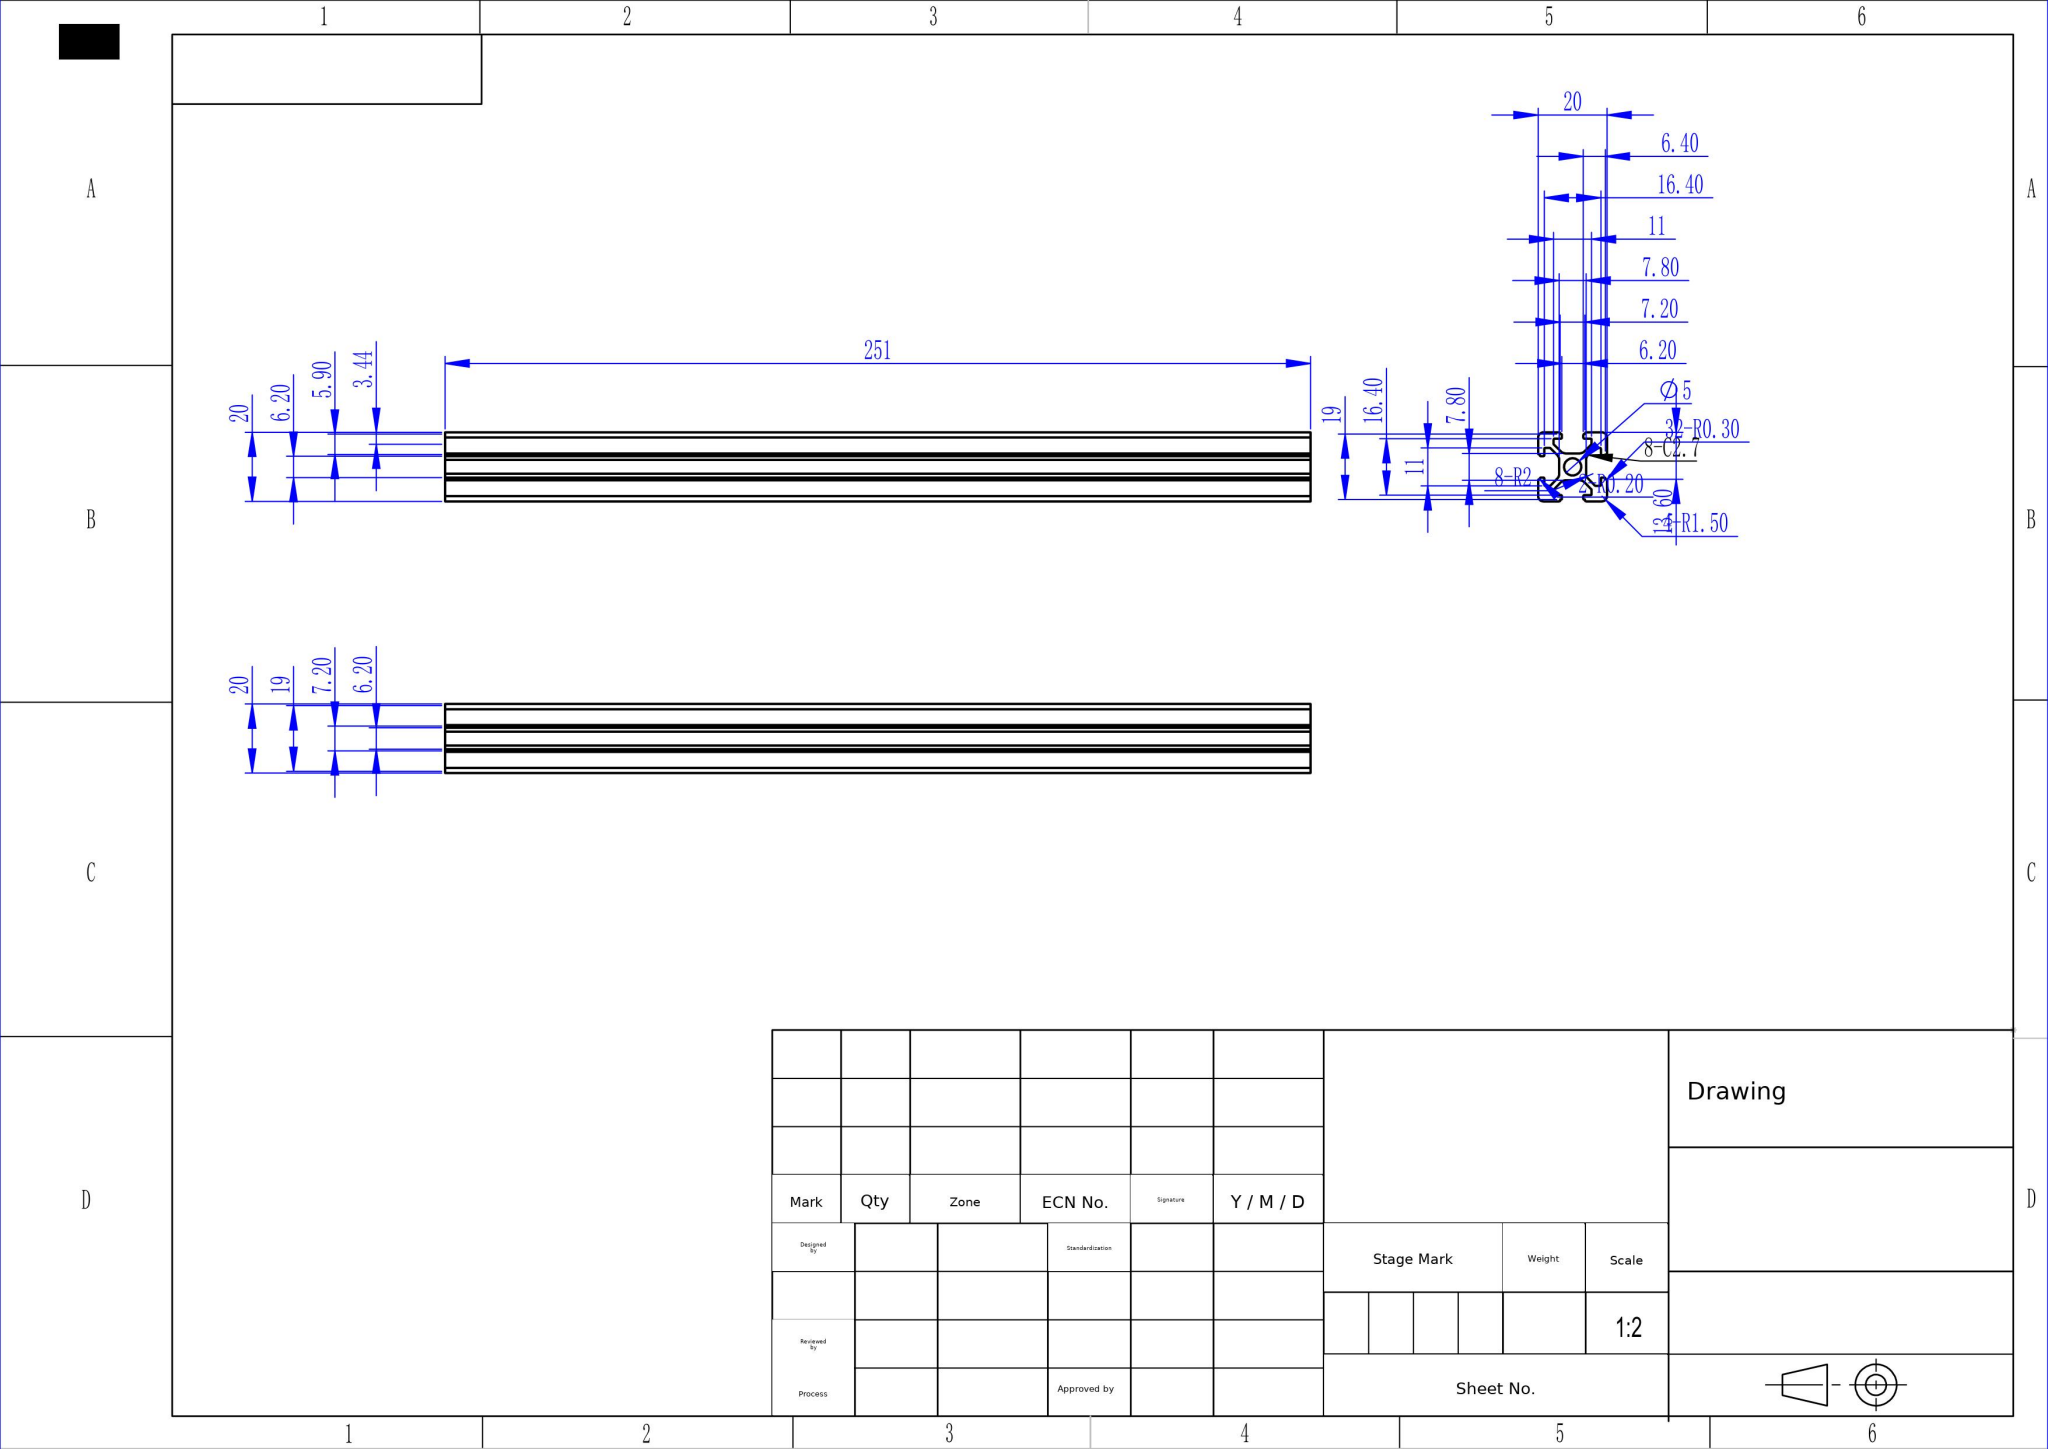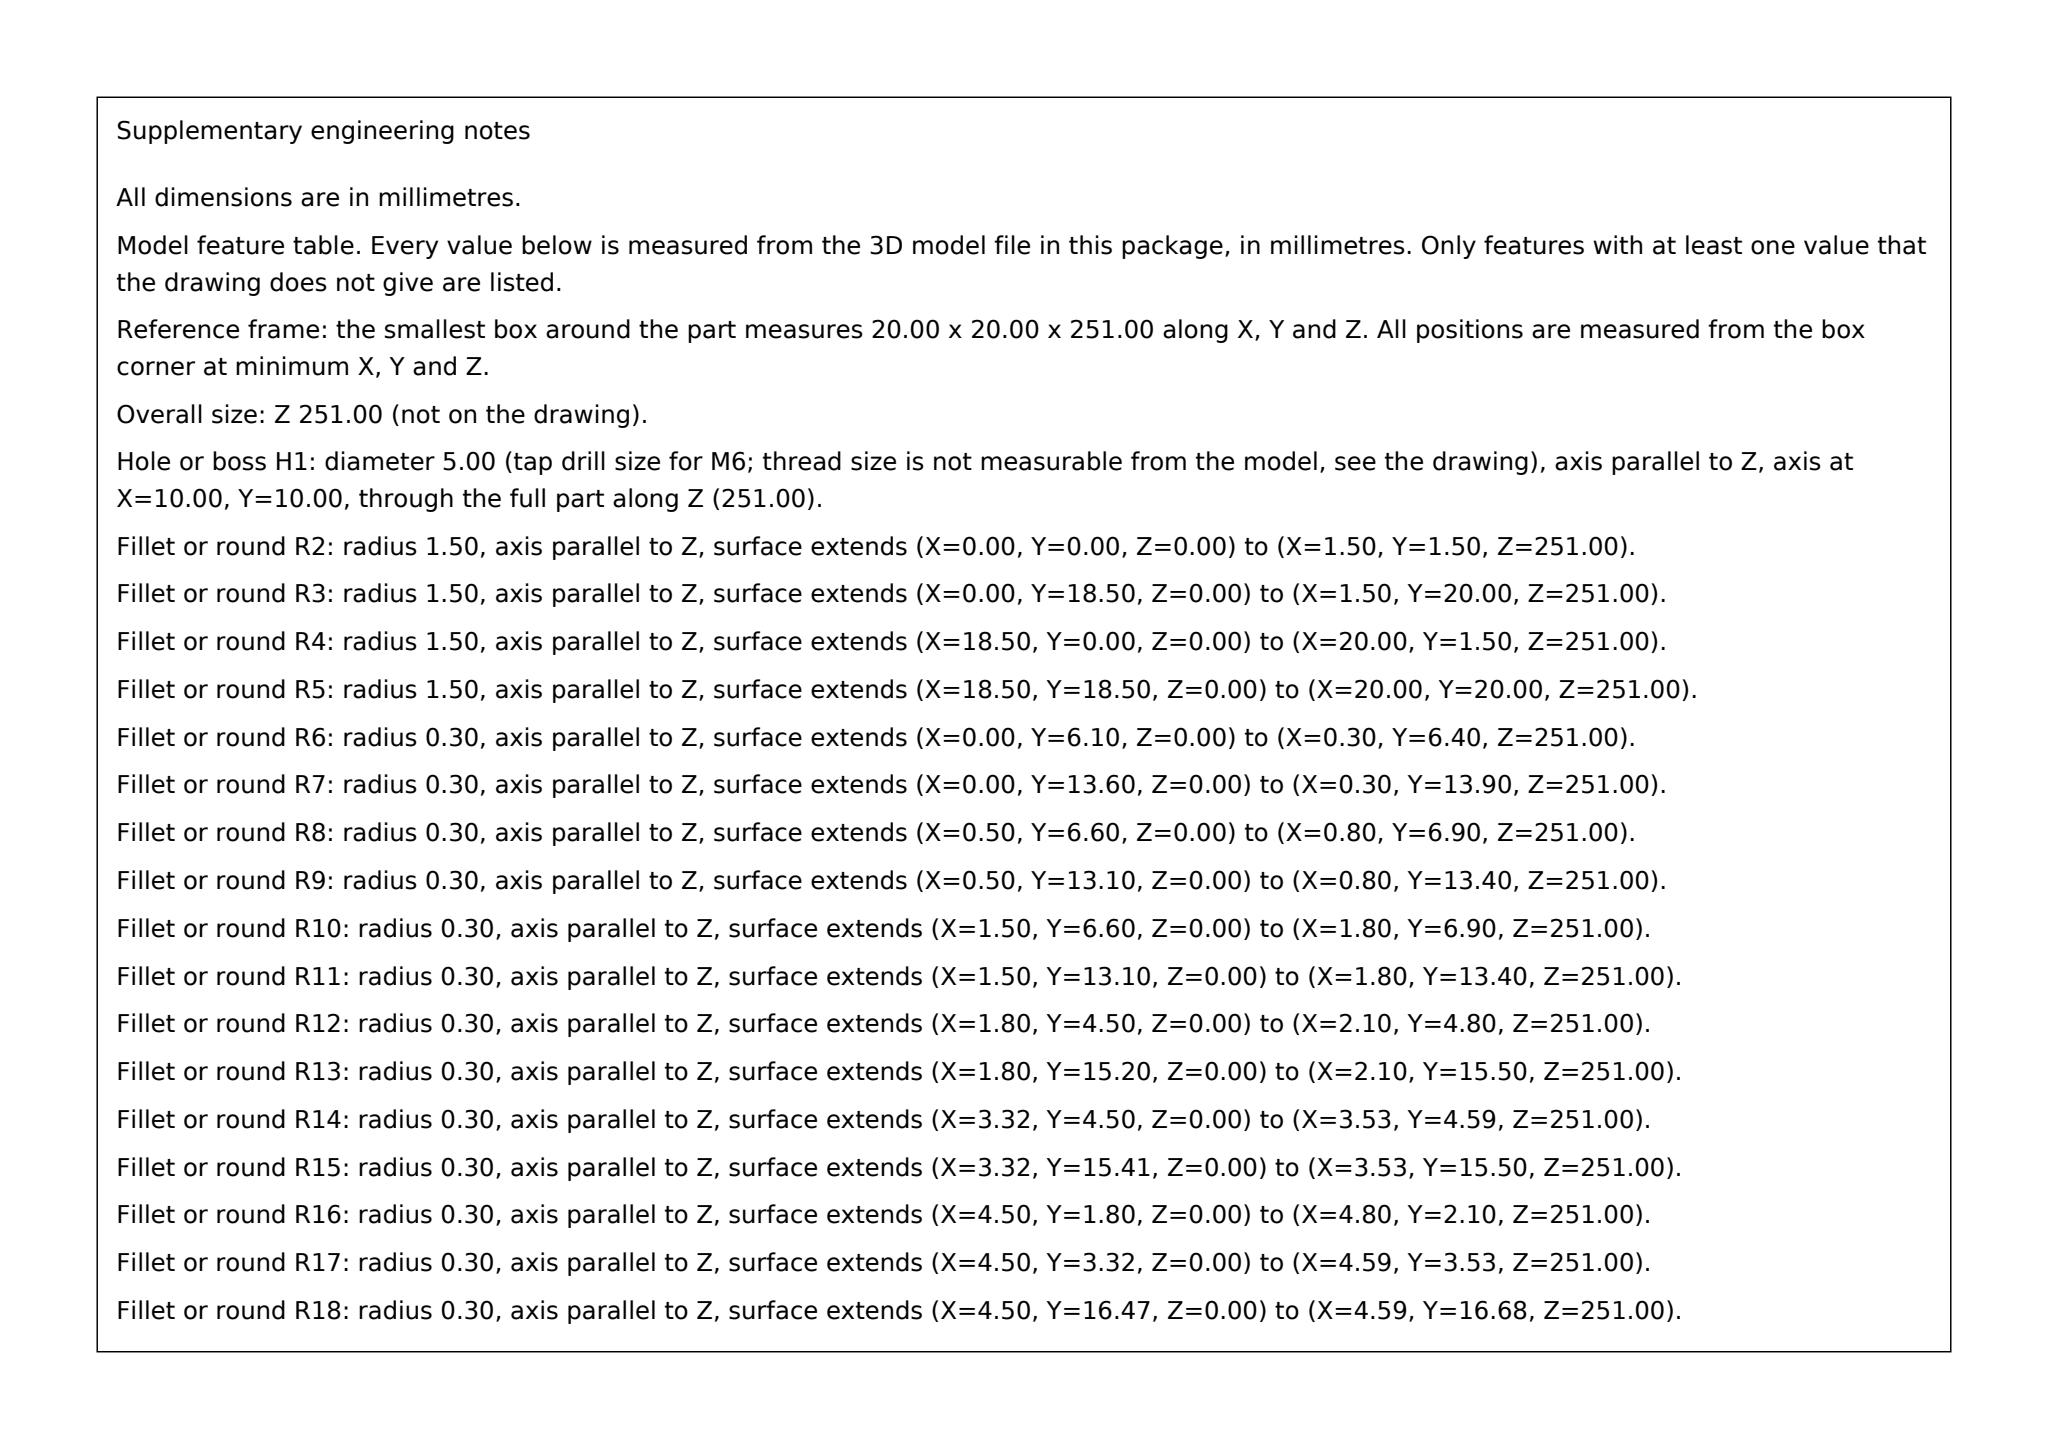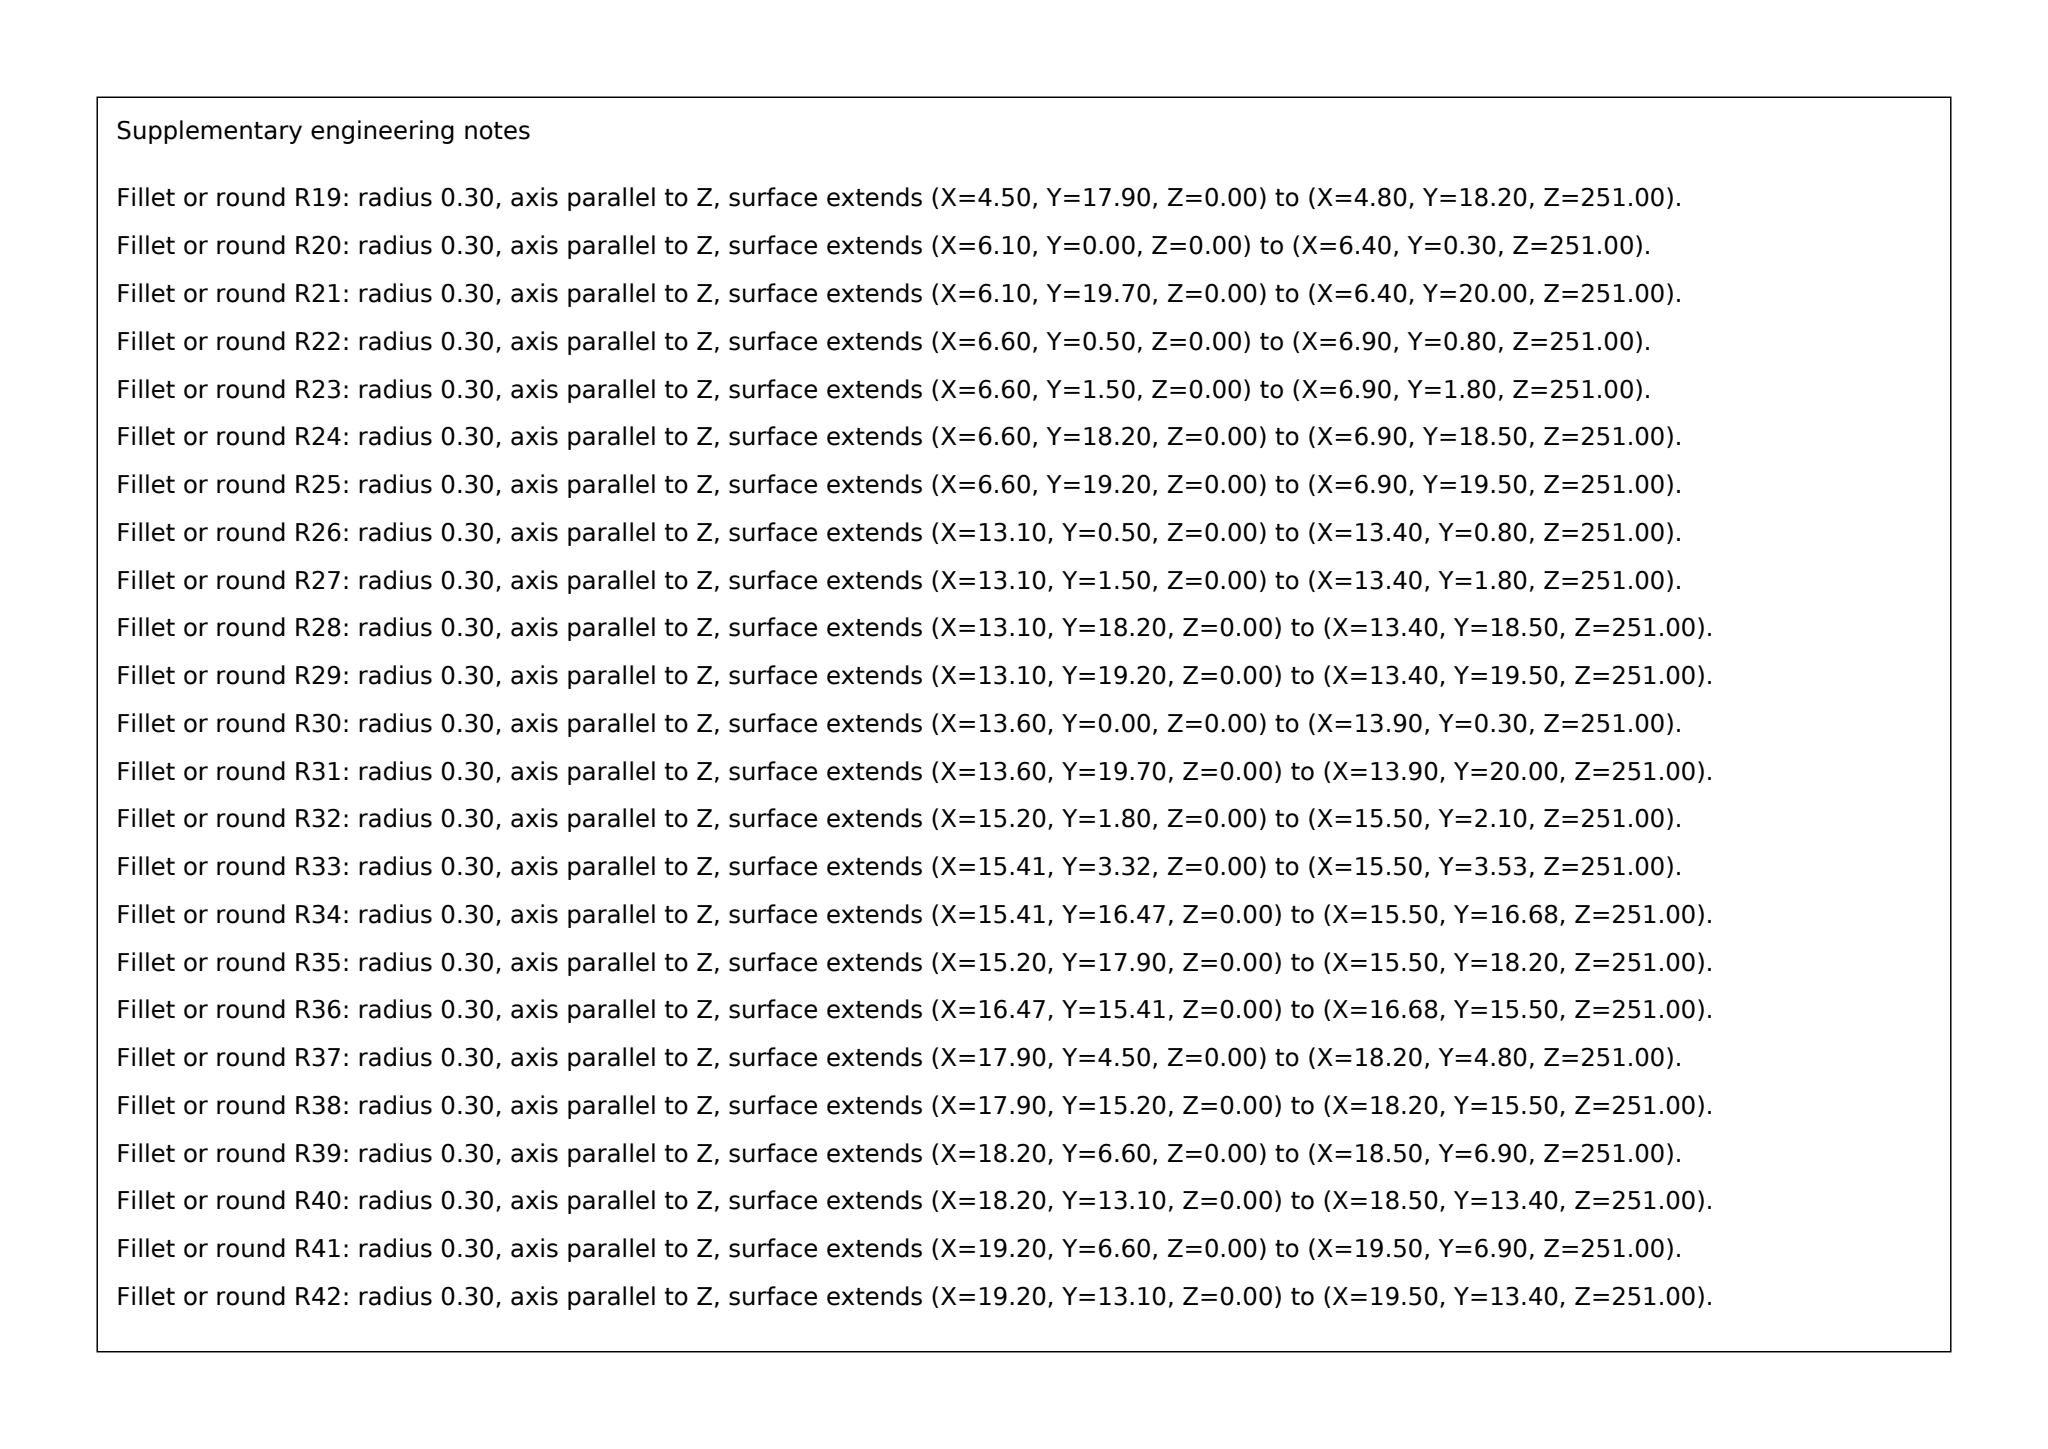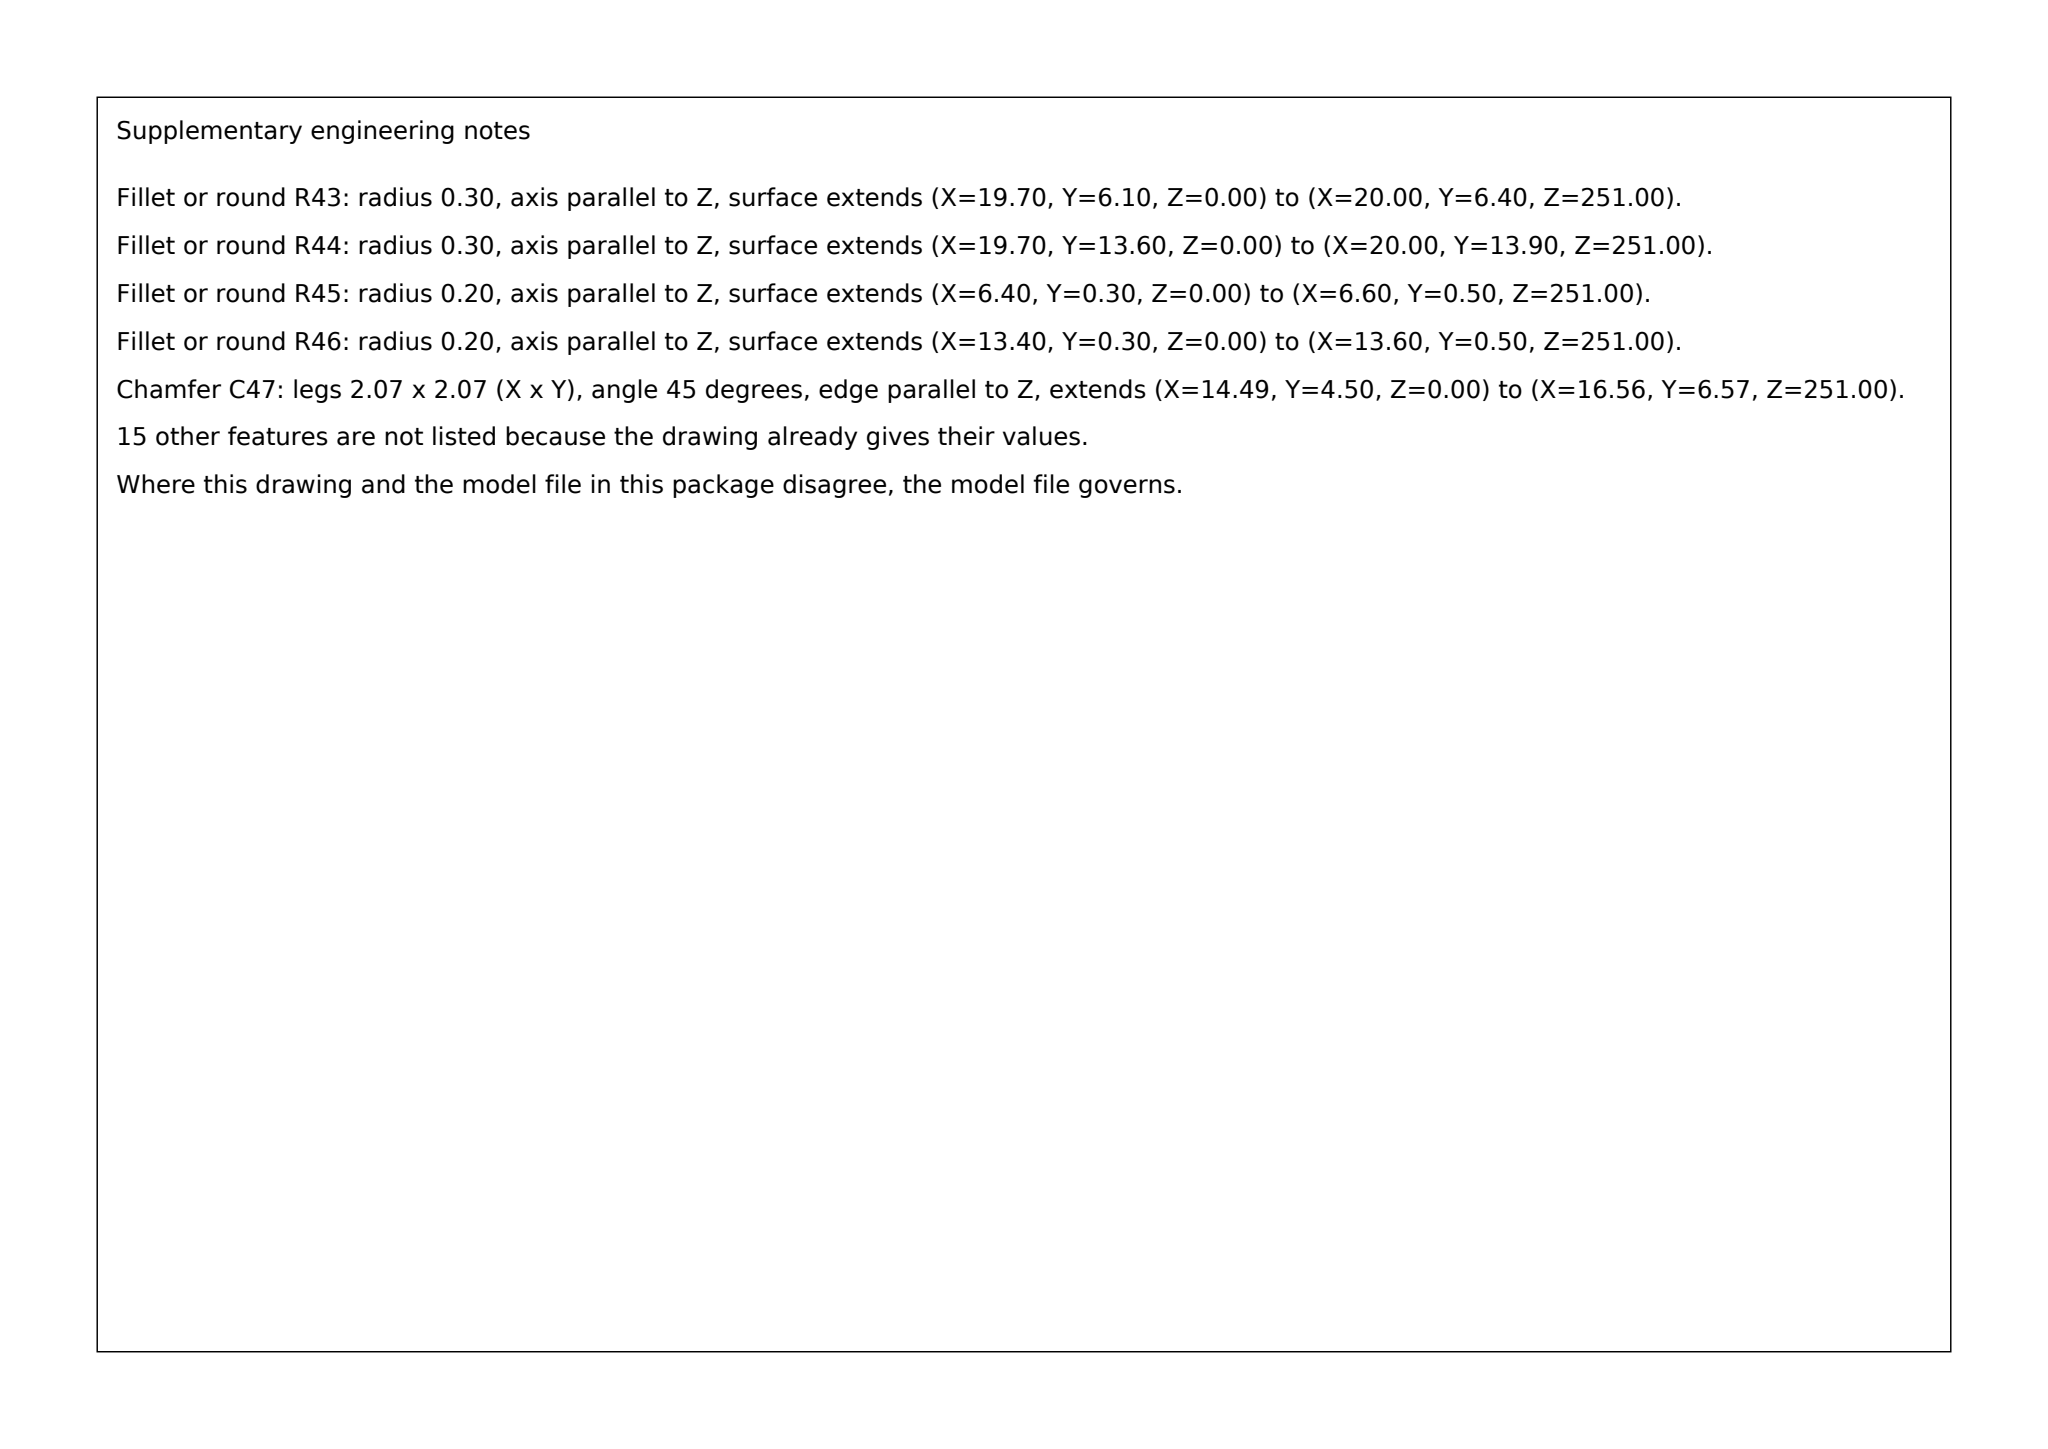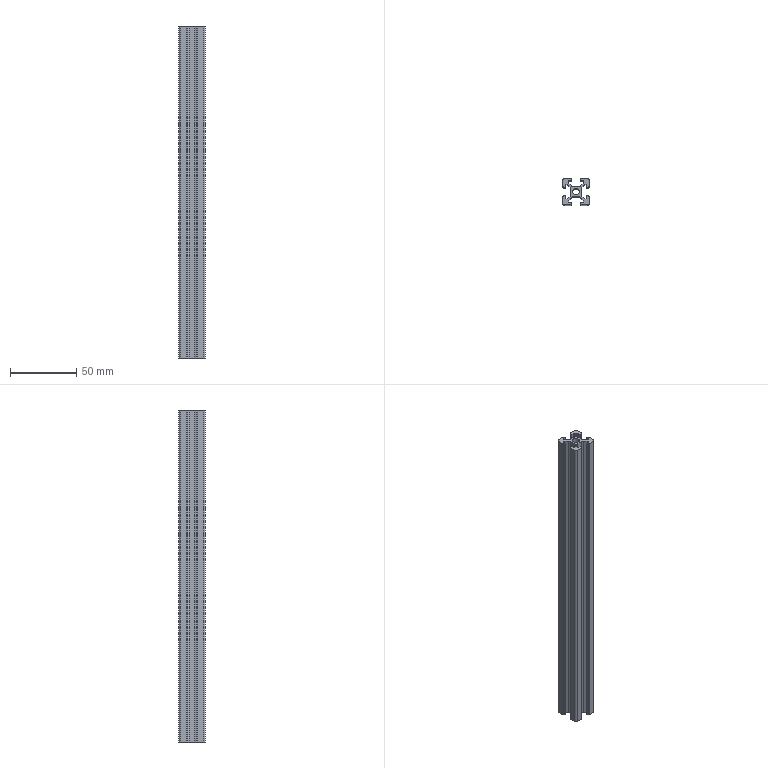Part | SolidWorks | mm | 1 solid | 113 faces | box 20 x 20 x 251 mm | volume 43001 mm3 | plane 58 | cylinder 55 | commonest cylinder face diameters 0.6 x39 4 x8 3 x4 5 x2 0.4 x2
build123d program:
from build123d import *

# Parameters (mm, degrees)
SKETCH1_R           = 2.5
BOSS_EXTRUDE1_DEPTH = 251


with BuildPart() as part:
    # Sketch1 → Boss-Extrude1 (new body)
    with BuildSketch(Plane(origin=(0, 0, 0), x_dir=(-1, 0, 0), z_dir=(0, 0, -1))):
        with BuildLine():
            Line((-5845.236, 2818.35), (-5845.236, 2820.15))
            ThreePointArc((-5845.236, 2820.15), (-5845.323, 2820.362), (-5845.536, 2820.45))
            Line((-5845.536, 2820.45), (-5846.236, 2820.45))
            ThreePointArc((-5846.236, 2820.45), (-5846.448, 2820.362), (-5846.536, 2820.15))
            Line((-5846.536, 2820.15), (-5846.536, 2819.95))
            Line((-5846.536, 2819.95), (-5846.736, 2819.95))
            ThreePointArc((-5846.736, 2819.95), (-5846.948, 2819.862), (-5847.036, 2819.65))
            Line((-5847.036, 2819.65), (-5847.036, 2815.05))
            ThreePointArc((-5847.036, 2815.05), (-5846.596, 2813.989), (-5845.536, 2813.55))
            Line((-5845.536, 2813.55), (-5840.936, 2813.55))
            ThreePointArc((-5840.936, 2813.55), (-5840.723, 2813.638), (-5840.636, 2813.85))
            ThreePointArc((-5840.636, 2813.85), (-5840.577, 2813.991), (-5840.436, 2814.05))
            ThreePointArc((-5840.436, 2814.05), (-5840.223, 2814.138), (-5840.136, 2814.35))
            Line((-5840.136, 2814.35), (-5840.136, 2815.05))
            ThreePointArc((-5840.136, 2815.05), (-5840.223, 2815.262), (-5840.436, 2815.35))
            Line((-5840.436, 2815.35), (-5842.236, 2815.35))
            ThreePointArc((-5842.236, 2815.35), (-5842.448, 2815.438), (-5842.536, 2815.65))
            Line((-5842.536, 2815.65), (-5842.536, 2816.865))
            ThreePointArc((-5842.536, 2816.865), (-5842.513, 2816.98), (-5842.448, 2817.077))
            Line((-5842.448, 2817.077), (-5840.461, 2819.064))
            ThreePointArc((-5840.461, 2819.064), (-5839.812, 2819.498), (-5839.046, 2819.65))
            Line((-5839.046, 2819.65), (-5835.025, 2819.65))
            ThreePointArc((-5835.025, 2819.65), (-5834.259, 2819.498), (-5833.61, 2819.064))
            Line((-5833.61, 2819.064), (-5831.623, 2817.077))
            ThreePointArc((-5831.623, 2817.077), (-5831.558, 2816.98), (-5831.536, 2816.865))
            Line((-5831.536, 2816.865), (-5831.536, 2815.65))
            ThreePointArc((-5831.536, 2815.65), (-5831.623, 2815.438), (-5831.836, 2815.35))
            Line((-5831.836, 2815.35), (-5833.636, 2815.35))
            ThreePointArc((-5833.636, 2815.35), (-5833.848, 2815.262), (-5833.936, 2815.05))
            Line((-5833.936, 2815.05), (-5833.936, 2814.35))
            ThreePointArc((-5833.936, 2814.35), (-5833.848, 2814.138), (-5833.636, 2814.05))
            ThreePointArc((-5833.636, 2814.05), (-5833.494, 2813.991), (-5833.436, 2813.85))
            ThreePointArc((-5833.436, 2813.85), (-5833.348, 2813.638), (-5833.136, 2813.55))
            Line((-5833.136, 2813.55), (-5828.536, 2813.55))
            ThreePointArc((-5828.536, 2813.55), (-5827.475, 2813.989), (-5827.036, 2815.05))
            Line((-5827.036, 2815.05), (-5827.036, 2819.65))
            ThreePointArc((-5827.036, 2819.65), (-5827.123, 2819.862), (-5827.336, 2819.95))
            Line((-5827.336, 2819.95), (-5827.536, 2819.95))
            Line((-5827.536, 2819.95), (-5827.536, 2820.15))
            ThreePointArc((-5827.536, 2820.15), (-5827.623, 2820.362), (-5827.836, 2820.45))
            Line((-5827.836, 2820.45), (-5828.536, 2820.45))
            ThreePointArc((-5828.536, 2820.45), (-5828.748, 2820.362), (-5828.836, 2820.15))
            Line((-5828.836, 2820.15), (-5828.836, 2818.35))
            ThreePointArc((-5828.836, 2818.35), (-5828.923, 2818.138), (-5829.136, 2818.05))
            Line((-5829.136, 2818.05), (-5830.351, 2818.05))
            ThreePointArc((-5830.351, 2818.05), (-5830.465, 2818.073), (-5830.563, 2818.138))
            Line((-5830.563, 2818.138), (-5832.55, 2820.125))
            ThreePointArc((-5832.55, 2820.125), (-5832.983, 2820.774), (-5833.136, 2821.539))
            Line((-5833.136, 2821.539), (-5833.136, 2825.561))
            ThreePointArc((-5833.136, 2825.561), (-5832.983, 2826.326), (-5832.55, 2826.975))
            Line((-5832.55, 2826.975), (-5830.563, 2828.962))
            ThreePointArc((-5830.563, 2828.962), (-5830.465, 2829.027), (-5830.351, 2829.05))
            Line((-5830.351, 2829.05), (-5829.136, 2829.05))
            ThreePointArc((-5829.136, 2829.05), (-5828.923, 2828.962), (-5828.836, 2828.75))
            Line((-5828.836, 2828.75), (-5828.836, 2826.95))
            ThreePointArc((-5828.836, 2826.95), (-5828.748, 2826.738), (-5828.536, 2826.65))
            Line((-5828.536, 2826.65), (-5827.836, 2826.65))
            ThreePointArc((-5827.836, 2826.65), (-5827.623, 2826.738), (-5827.536, 2826.95))
            Line((-5827.536, 2826.95), (-5827.536, 2827.15))
            Line((-5827.536, 2827.15), (-5827.336, 2827.15))
            ThreePointArc((-5827.336, 2827.15), (-5827.123, 2827.238), (-5827.036, 2827.45))
            Line((-5827.036, 2827.45), (-5827.036, 2832.05))
            ThreePointArc((-5827.036, 2832.05), (-5827.475, 2833.11), (-5828.536, 2833.55))
            Line((-5828.536, 2833.55), (-5833.136, 2833.55))
            ThreePointArc((-5833.136, 2833.55), (-5833.348, 2833.462), (-5833.436, 2833.25))
            Line((-5833.436, 2833.25), (-5833.436, 2833.05))
            Line((-5833.436, 2833.05), (-5833.636, 2833.05))
            ThreePointArc((-5833.636, 2833.05), (-5833.848, 2832.962), (-5833.936, 2832.75))
            Line((-5833.936, 2832.75), (-5833.936, 2832.05))
            ThreePointArc((-5833.936, 2832.05), (-5833.848, 2831.838), (-5833.636, 2831.75))
            Line((-5833.636, 2831.75), (-5831.836, 2831.75))
            ThreePointArc((-5831.836, 2831.75), (-5831.623, 2831.662), (-5831.536, 2831.45))
            Line((-5831.536, 2831.45), (-5831.536, 2830.235))
            ThreePointArc((-5831.536, 2830.235), (-5831.558, 2830.12), (-5831.623, 2830.023))
            Line((-5831.623, 2830.023), (-5833.61, 2828.036))
            ThreePointArc((-5833.61, 2828.036), (-5834.259, 2827.602), (-5835.025, 2827.45))
            Line((-5835.025, 2827.45), (-5839.046, 2827.45))
            ThreePointArc((-5839.046, 2827.45), (-5839.812, 2827.602), (-5840.461, 2828.036))
            Line((-5840.461, 2828.036), (-5842.448, 2830.023))
            ThreePointArc((-5842.448, 2830.023), (-5842.513, 2830.12), (-5842.536, 2830.235))
            Line((-5842.536, 2830.235), (-5842.536, 2831.45))
            ThreePointArc((-5842.536, 2831.45), (-5842.448, 2831.662), (-5842.236, 2831.75))
            Line((-5842.236, 2831.75), (-5840.436, 2831.75))
            ThreePointArc((-5840.436, 2831.75), (-5840.223, 2831.838), (-5840.136, 2832.05))
            Line((-5840.136, 2832.05), (-5840.136, 2832.75))
            ThreePointArc((-5840.136, 2832.75), (-5840.223, 2832.962), (-5840.436, 2833.05))
            Line((-5840.436, 2833.05), (-5840.636, 2833.05))
            Line((-5840.636, 2833.05), (-5840.636, 2833.25))
            ThreePointArc((-5840.636, 2833.25), (-5840.723, 2833.462), (-5840.936, 2833.55))
            Line((-5840.936, 2833.55), (-5845.536, 2833.55))
            ThreePointArc((-5845.536, 2833.55), (-5846.596, 2833.11), (-5847.036, 2832.05))
            Line((-5847.036, 2832.05), (-5847.036, 2827.45))
            ThreePointArc((-5847.036, 2827.45), (-5846.948, 2827.238), (-5846.736, 2827.15))
            Line((-5846.736, 2827.15), (-5846.536, 2827.15))
            Line((-5846.536, 2827.15), (-5846.536, 2826.95))
            ThreePointArc((-5846.536, 2826.95), (-5846.448, 2826.738), (-5846.236, 2826.65))
            Line((-5846.236, 2826.65), (-5845.536, 2826.65))
            ThreePointArc((-5845.536, 2826.65), (-5845.323, 2826.738), (-5845.236, 2826.95))
            Line((-5845.236, 2826.95), (-5845.236, 2828.75))
            ThreePointArc((-5845.236, 2828.75), (-5845.148, 2828.962), (-5844.936, 2829.05))
            Line((-5844.936, 2829.05), (-5843.72, 2829.05))
            ThreePointArc((-5843.72, 2829.05), (-5843.606, 2829.027), (-5843.508, 2828.962))
            Line((-5843.508, 2828.962), (-5841.521, 2826.975))
            ThreePointArc((-5841.521, 2826.975), (-5841.088, 2826.326), (-5840.936, 2825.561))
            Line((-5840.936, 2825.561), (-5840.936, 2821.539))
            ThreePointArc((-5840.936, 2821.539), (-5841.088, 2820.774), (-5841.521, 2820.125))
            Line((-5841.521, 2820.125), (-5843.596, 2818.05))
            Line((-5843.596, 2818.05), (-5844.936, 2818.05))
            ThreePointArc((-5844.936, 2818.05), (-5845.148, 2818.138), (-5845.236, 2818.35))
        make_face()
        with Locations(Location((-5837.036, 2823.55, 0), (0, 0, 180))):
            Circle(SKETCH1_R, mode=Mode.SUBTRACT)
    extrude(amount=-BOSS_EXTRUDE1_DEPTH)


solid = part.part